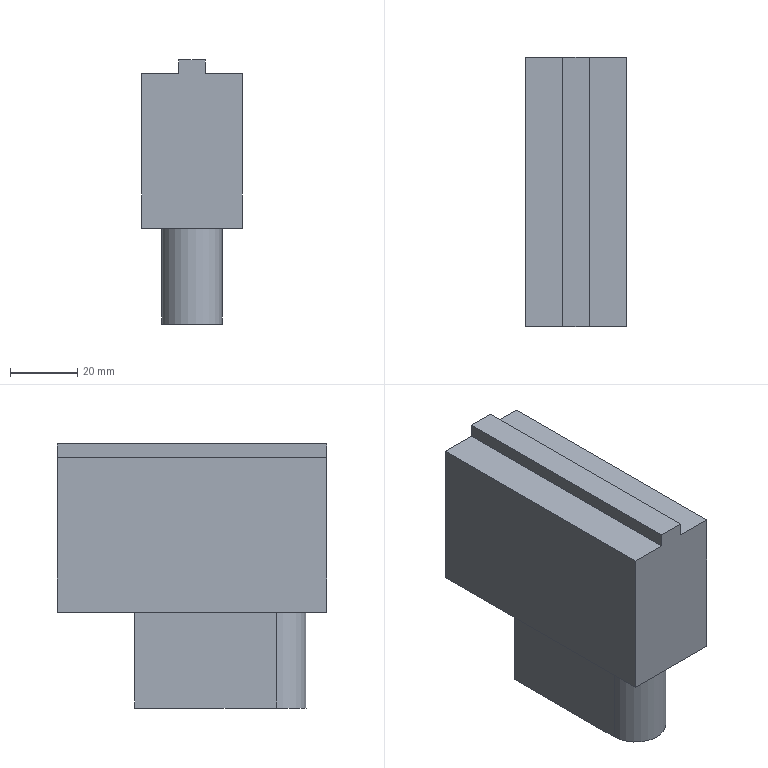Component | SolidWorks | 12AOuterSideWheel-EngravingAndMillingAxis-1_12AOuterSideWheelSeat-1 | 1 solid | 29 faces | box 30 x 80 x 78.5 mm | volume 131688 mm3 | plane 17 | cylinder 8 | cone 4 | commonest cylinder face diameters 8.5 x4 12.5 x3 18 x1 | material Cr12MoV
build123d program:
from build123d import *

# Parameters (mm, degrees)
SKETCH1_W              = 80
SKETCH1_H              = 46
BOSS_EXTRUDE1_DEPTH    = 30
SKETCH2_W              = 80
SKETCH2_H              = 8
BOSS_EXTRUDE2_DEPTH    = 4
BOSS_EXTRUDE3_DEPTH    = 28.5
M10_TAPPED_HOLE1_D     = 8.5
M10_TAPPED_HOLE1_DEPTH = 25
M10_TAPPED_HOLE1_TIP   = 2.554
CUT_EXTRUDE1_DEPTH     = 24


with BuildPart() as part:
    # Sketch1 → Boss-Extrude1 (new body)
    with BuildSketch(Plane.XY):
        with Locations((40, -23)):
            Rectangle(SKETCH1_W, SKETCH1_H)
    extrude(amount=BOSS_EXTRUDE1_DEPTH)

    # Sketch2 → Boss-Extrude2 (add)
    with BuildSketch(Plane(origin=(0, 0, 0), x_dir=(1, 0, 0), z_dir=(0, 1, 0))):
        with Locations((40, -15)):
            Rectangle(SKETCH2_W, SKETCH2_H)
    extrude(amount=BOSS_EXTRUDE2_DEPTH)

    # Sketch3 → Boss-Extrude3 (add)
    with BuildSketch(Plane.XZ.offset(46)):
        with BuildLine():
            Line((57, 24), (57, 6))
            Line((57, 6), (15, 6))
            ThreePointArc((15, 6), (6, 15), (15, 24))
            Line((15, 24), (57, 24))
        make_face()
    extrude(amount=BOSS_EXTRUDE3_DEPTH)

    # M10 Tapped Hole1
    with Locations(Plane(origin=(0, -74.5, 0), x_dir=(-1, 0, 0), z_dir=(0, -1, 0))):
        with Locations((-35, -15), (-15, -15)):
            Hole(M10_TAPPED_HOLE1_D / 2, depth=M10_TAPPED_HOLE1_DEPTH)
            with Locations((0, 0, -(M10_TAPPED_HOLE1_DEPTH + M10_TAPPED_HOLE1_TIP / 2))):  # 118° drill point
                Cone(0, M10_TAPPED_HOLE1_D / 2, M10_TAPPED_HOLE1_TIP, mode=Mode.SUBTRACT)

    # Sketch6 → Cut-Extrude1 (cut)
    with BuildSketch(Plane.XZ.offset(74.5)):
        with BuildLine():
            Line((57, 19.25), (53.083, 19.25))
            ThreePointArc((53.083, 19.25), (42.25, 15), (53.083, 10.75))
            Line((53.083, 10.75), (57, 10.75))
            Line((57, 10.75), (57, 19.25))
        make_face()
    extrude(amount=-CUT_EXTRUDE1_DEPTH, mode=Mode.SUBTRACT)


solid = part.part

# Placed as in the assembly
solid = solid.moved(Location((196.598, 111.538, 60.25), (90, 90, 0)))
STEP:
#1=COLOUR_RGB('',0.7922,0.8196,0.9333);
#2=FILL_AREA_STYLE_COLOUR('',#1);
#3=FILL_AREA_STYLE('',(#2));
#4=SURFACE_STYLE_FILL_AREA(#3);
#5=SURFACE_SIDE_STYLE('',(#4));
#6=SURFACE_STYLE_USAGE(.BOTH.,#5);
#7=PRESENTATION_STYLE_ASSIGNMENT((#6));
#8=CARTESIAN_POINT('',(8.577,6.301,0.3839));
#9=VERTEX_POINT('',#8);
#10=CARTESIAN_POINT('',(8.085,6.301,0.3839));
#11=VERTEX_POINT('',#10);
#12=CARTESIAN_POINT('',(8.331,6.301,0.3839));
#13=DIRECTION('',(0.,0.,-1.));
#14=DIRECTION('',(-1.,0.,0.));
#15=AXIS2_PLACEMENT_3D('',#12,#13,#14);
#16=CIRCLE('',#15,0.2461);
#17=EDGE_CURVE('',#9,#11,#16,.T.);
#18=ORIENTED_EDGE('',*,*,#17,.F.);
#19=CARTESIAN_POINT('',(8.577,6.301,-0.561));
#20=VERTEX_POINT('',#19);
#21=CARTESIAN_POINT('',(8.577,6.301,0.3839));
#22=DIRECTION('',(0.,0.,-1.));
#23=VECTOR('',#22,39.37);
#24=LINE('',#21,#23);
#25=EDGE_CURVE('',#9,#20,#24,.T.);
#26=ORIENTED_EDGE('',*,*,#25,.T.);
#27=CARTESIAN_POINT('',(8.085,6.301,-0.561));
#28=VERTEX_POINT('',#27);
#29=CARTESIAN_POINT('',(8.331,6.301,-0.561));
#30=DIRECTION('',(0.,0.,-1.));
#31=DIRECTION('',(-1.,0.,0.));
#32=AXIS2_PLACEMENT_3D('',#29,#30,#31);
#33=CIRCLE('',#32,0.2461);
#34=EDGE_CURVE('',#20,#28,#33,.T.);
#35=ORIENTED_EDGE('',*,*,#34,.T.);
#36=CARTESIAN_POINT('',(8.085,6.301,0.3839));
#37=DIRECTION('',(0.,0.,-1.));
#38=VECTOR('',#37,39.37);
#39=LINE('',#36,#38);
#40=EDGE_CURVE('',#11,#28,#39,.T.);
#41=ORIENTED_EDGE('',*,*,#40,.F.);
#42=EDGE_LOOP('',(#18,#26,#35,#41));
#43=FACE_OUTER_BOUND('',#42,.T.);
#44=CARTESIAN_POINT('',(8.331,6.301,0.3839));
#45=DIRECTION('',(0.,0.,-1.));
#46=DIRECTION('',(-1.,0.,0.));
#47=AXIS2_PLACEMENT_3D('',#44,#45,#46);
#48=CYLINDRICAL_SURFACE('',#47,0.2461);
#49=ADVANCED_FACE('',(#43),#48,.F.);
#50=CARTESIAN_POINT('',(8.163,6.481,0.3839));
#51=VERTEX_POINT('',#50);
#52=CARTESIAN_POINT('',(8.331,6.301,0.3839));
#53=DIRECTION('',(0.,0.,-1.));
#54=DIRECTION('',(-1.,0.,0.));
#55=AXIS2_PLACEMENT_3D('',#52,#53,#54);
#56=CIRCLE('',#55,0.2461);
#57=EDGE_CURVE('',#11,#51,#56,.T.);
#58=ORIENTED_EDGE('',*,*,#57,.F.);
#59=ORIENTED_EDGE('',*,*,#40,.T.);
#60=CARTESIAN_POINT('',(8.163,6.481,-0.561));
#61=VERTEX_POINT('',#60);
#62=CARTESIAN_POINT('',(8.331,6.301,-0.561));
#63=DIRECTION('',(0.,0.,-1.));
#64=DIRECTION('',(-1.,0.,0.));
#65=AXIS2_PLACEMENT_3D('',#62,#63,#64);
#66=CIRCLE('',#65,0.2461);
#67=EDGE_CURVE('',#28,#61,#66,.T.);
#68=ORIENTED_EDGE('',*,*,#67,.T.);
#69=CARTESIAN_POINT('',(8.163,6.481,0.3839));
#70=DIRECTION('',(0.,0.,-1.));
#71=VECTOR('',#70,39.37);
#72=LINE('',#69,#71);
#73=EDGE_CURVE('',#51,#61,#72,.T.);
#74=ORIENTED_EDGE('',*,*,#73,.F.);
#75=EDGE_LOOP('',(#58,#59,#68,#74));
#76=FACE_OUTER_BOUND('',#75,.T.);
#77=CARTESIAN_POINT('',(8.331,6.301,0.3839));
#78=DIRECTION('',(0.,0.,-1.));
#79=DIRECTION('',(-1.,0.,0.));
#80=AXIS2_PLACEMENT_3D('',#77,#78,#79);
#81=CYLINDRICAL_SURFACE('',#80,0.2461);
#82=ADVANCED_FACE('',(#76),#81,.F.);
#83=CARTESIAN_POINT('',(8.498,4.982,0.4232));
#84=VERTEX_POINT('',#83);
#85=CARTESIAN_POINT('',(8.163,4.982,0.4232));
#86=VERTEX_POINT('',#85);
#87=CARTESIAN_POINT('',(8.331,4.982,0.4232));
#88=DIRECTION('',(0.,0.,-1.));
#89=DIRECTION('',(-1.,0.,0.));
#90=AXIS2_PLACEMENT_3D('',#87,#88,#89);
#91=CIRCLE('',#90,0.1673);
#92=EDGE_CURVE('',#84,#86,#91,.T.);
#93=ORIENTED_EDGE('',*,*,#92,.F.);
#94=CARTESIAN_POINT('',(8.498,4.982,-0.561));
#95=VERTEX_POINT('',#94);
#96=CARTESIAN_POINT('',(8.498,4.982,-0.561));
#97=DIRECTION('',(0.,0.,-1.));
#98=VECTOR('',#97,39.37);
#99=LINE('',#96,#98);
#100=EDGE_CURVE('',#84,#95,#99,.T.);
#101=ORIENTED_EDGE('',*,*,#100,.T.);
#102=CARTESIAN_POINT('',(8.163,4.982,-0.561));
#103=VERTEX_POINT('',#102);
#104=CARTESIAN_POINT('',(8.331,4.982,-0.561));
#105=DIRECTION('',(0.,0.,-1.));
#106=DIRECTION('',(-1.,0.,0.));
#107=AXIS2_PLACEMENT_3D('',#104,#105,#106);
#108=CIRCLE('',#107,0.1673);
#109=EDGE_CURVE('',#95,#103,#108,.T.);
#110=ORIENTED_EDGE('',*,*,#109,.T.);
#111=CARTESIAN_POINT('',(8.163,4.982,-0.561));
#112=DIRECTION('',(0.,0.,-1.));
#113=VECTOR('',#112,39.37);
#114=LINE('',#111,#113);
#115=EDGE_CURVE('',#86,#103,#114,.T.);
#116=ORIENTED_EDGE('',*,*,#115,.F.);
#117=EDGE_LOOP('',(#93,#101,#110,#116));
#118=FACE_OUTER_BOUND('',#117,.T.);
#119=CARTESIAN_POINT('',(8.331,4.982,-0.561));
#120=DIRECTION('',(0.,0.,-1.));
#121=DIRECTION('',(-1.,0.,0.));
#122=AXIS2_PLACEMENT_3D('',#119,#120,#121);
#123=CYLINDRICAL_SURFACE('',#122,0.1673);
#124=ADVANCED_FACE('',(#118),#123,.F.);
#125=CARTESIAN_POINT('',(8.331,4.982,0.5238));
#126=VERTEX_POINT('',#125);
#127=CARTESIAN_POINT('',(8.163,4.982,0.4232));
#128=DIRECTION('',(-0.8572,0.,-0.515));
#129=VECTOR('',#128,39.37);
#130=LINE('',#127,#129);
#131=EDGE_CURVE('',#126,#86,#130,.T.);
#132=ORIENTED_EDGE('',*,*,#131,.F.);
#133=CARTESIAN_POINT('',(8.498,4.982,0.4232));
#134=DIRECTION('',(0.8572,0.,-0.515));
#135=VECTOR('',#134,39.37);
#136=LINE('',#133,#135);
#137=EDGE_CURVE('',#126,#84,#136,.T.);
#138=ORIENTED_EDGE('',*,*,#137,.T.);
#139=ORIENTED_EDGE('',*,*,#92,.T.);
#140=EDGE_LOOP('',(#132,#138,#139));
#141=FACE_OUTER_BOUND('',#140,.T.);
#142=CARTESIAN_POINT('',(8.331,4.982,0.4232));
#143=DIRECTION('',(0.,0.,-1.));
#144=DIRECTION('',(-1.,0.,0.));
#145=AXIS2_PLACEMENT_3D('',#142,#143,#144);
#146=CONICAL_SURFACE('',#145,0.1673,1.03);
#147=ADVANCED_FACE('',(#141),#146,.F.);
#148=CARTESIAN_POINT('',(8.498,5.769,0.4232));
#149=VERTEX_POINT('',#148);
#150=CARTESIAN_POINT('',(8.163,5.769,0.4232));
#151=VERTEX_POINT('',#150);
#152=CARTESIAN_POINT('',(8.331,5.769,0.4232));
#153=DIRECTION('',(0.,0.,-1.));
#154=DIRECTION('',(-1.,0.,0.));
#155=AXIS2_PLACEMENT_3D('',#152,#153,#154);
#156=CIRCLE('',#155,0.1673);
#157=EDGE_CURVE('',#149,#151,#156,.T.);
#158=ORIENTED_EDGE('',*,*,#157,.F.);
#159=CARTESIAN_POINT('',(8.498,5.769,-0.561));
#160=VERTEX_POINT('',#159);
#161=CARTESIAN_POINT('',(8.498,5.769,-0.561));
#162=DIRECTION('',(0.,0.,-1.));
#163=VECTOR('',#162,39.37);
#164=LINE('',#161,#163);
#165=EDGE_CURVE('',#149,#160,#164,.T.);
#166=ORIENTED_EDGE('',*,*,#165,.T.);
#167=CARTESIAN_POINT('',(8.163,5.769,-0.561));
#168=VERTEX_POINT('',#167);
#169=CARTESIAN_POINT('',(8.331,5.769,-0.561));
#170=DIRECTION('',(0.,0.,-1.));
#171=DIRECTION('',(-1.,0.,0.));
#172=AXIS2_PLACEMENT_3D('',#169,#170,#171);
#173=CIRCLE('',#172,0.1673);
#174=EDGE_CURVE('',#160,#168,#173,.T.);
#175=ORIENTED_EDGE('',*,*,#174,.T.);
#176=CARTESIAN_POINT('',(8.163,5.769,-0.561));
#177=DIRECTION('',(0.,0.,-1.));
#178=VECTOR('',#177,39.37);
#179=LINE('',#176,#178);
#180=EDGE_CURVE('',#151,#168,#179,.T.);
#181=ORIENTED_EDGE('',*,*,#180,.F.);
#182=EDGE_LOOP('',(#158,#166,#175,#181));
#183=FACE_OUTER_BOUND('',#182,.T.);
#184=CARTESIAN_POINT('',(8.331,5.769,-0.561));
#185=DIRECTION('',(0.,0.,-1.));
#186=DIRECTION('',(-1.,0.,0.));
#187=AXIS2_PLACEMENT_3D('',#184,#185,#186);
#188=CYLINDRICAL_SURFACE('',#187,0.1673);
#189=ADVANCED_FACE('',(#183),#188,.F.);
#190=CARTESIAN_POINT('',(8.331,5.769,0.5238));
#191=VERTEX_POINT('',#190);
#192=CARTESIAN_POINT('',(8.163,5.769,0.4232));
#193=DIRECTION('',(-0.8572,0.,-0.515));
#194=VECTOR('',#193,39.37);
#195=LINE('',#192,#194);
#196=EDGE_CURVE('',#191,#151,#195,.T.);
#197=ORIENTED_EDGE('',*,*,#196,.F.);
#198=CARTESIAN_POINT('',(8.498,5.769,0.4232));
#199=DIRECTION('',(0.8572,0.,-0.515));
#200=VECTOR('',#199,39.37);
#201=LINE('',#198,#200);
#202=EDGE_CURVE('',#191,#149,#201,.T.);
#203=ORIENTED_EDGE('',*,*,#202,.T.);
#204=ORIENTED_EDGE('',*,*,#157,.T.);
#205=EDGE_LOOP('',(#197,#203,#204));
#206=FACE_OUTER_BOUND('',#205,.T.);
#207=CARTESIAN_POINT('',(8.331,5.769,0.4232));
#208=DIRECTION('',(0.,0.,-1.));
#209=DIRECTION('',(-1.,0.,0.));
#210=AXIS2_PLACEMENT_3D('',#207,#208,#209);
#211=CONICAL_SURFACE('',#210,0.1673,1.03);
#212=ADVANCED_FACE('',(#206),#211,.F.);
#213=CARTESIAN_POINT('',(7.74,4.391,0.561));
#214=VERTEX_POINT('',#213);
#215=CARTESIAN_POINT('',(7.74,7.541,0.561));
#216=VERTEX_POINT('',#215);
#217=CARTESIAN_POINT('',(7.74,4.391,0.561));
#218=DIRECTION('',(0.,1.,0.));
#219=VECTOR('',#218,39.37);
#220=LINE('',#217,#219);
#221=EDGE_CURVE('',#214,#216,#220,.T.);
#222=ORIENTED_EDGE('',*,*,#221,.T.);
#223=CARTESIAN_POINT('',(8.921,7.541,0.561));
#224=VERTEX_POINT('',#223);
#225=CARTESIAN_POINT('',(8.921,7.541,0.561));
#226=DIRECTION('',(-1.,0.,0.));
#227=VECTOR('',#226,39.37);
#228=LINE('',#225,#227);
#229=EDGE_CURVE('',#224,#216,#228,.T.);
#230=ORIENTED_EDGE('',*,*,#229,.F.);
#231=CARTESIAN_POINT('',(8.921,4.391,0.561));
#232=VERTEX_POINT('',#231);
#233=CARTESIAN_POINT('',(8.921,4.391,0.561));
#234=DIRECTION('',(0.,1.,0.));
#235=VECTOR('',#234,39.37);
#236=LINE('',#233,#235);
#237=EDGE_CURVE('',#232,#224,#236,.T.);
#238=ORIENTED_EDGE('',*,*,#237,.F.);
#239=CARTESIAN_POINT('',(8.921,4.391,0.561));
#240=DIRECTION('',(-1.,0.,0.));
#241=VECTOR('',#240,39.37);
#242=LINE('',#239,#241);
#243=EDGE_CURVE('',#232,#214,#242,.T.);
#244=ORIENTED_EDGE('',*,*,#243,.T.);
#245=EDGE_LOOP('',(#222,#230,#238,#244));
#246=FACE_OUTER_BOUND('',#245,.T.);
#247=CARTESIAN_POINT('',(8.685,4.982,0.561));
#248=VERTEX_POINT('',#247);
#249=CARTESIAN_POINT('',(7.976,4.982,0.561));
#250=VERTEX_POINT('',#249);
#251=CARTESIAN_POINT('',(8.331,4.982,0.561));
#252=DIRECTION('',(0.,0.,-1.));
#253=DIRECTION('',(-1.,0.,0.));
#254=AXIS2_PLACEMENT_3D('',#251,#252,#253);
#255=CIRCLE('',#254,0.3543);
#256=EDGE_CURVE('',#248,#250,#255,.T.);
#257=ORIENTED_EDGE('',*,*,#256,.F.);
#258=CARTESIAN_POINT('',(8.685,6.635,0.561));
#259=VERTEX_POINT('',#258);
#260=CARTESIAN_POINT('',(8.685,4.982,0.561));
#261=DIRECTION('',(0.,-1.,0.));
#262=VECTOR('',#261,39.37);
#263=LINE('',#260,#262);
#264=EDGE_CURVE('',#259,#248,#263,.T.);
#265=ORIENTED_EDGE('',*,*,#264,.F.);
#266=CARTESIAN_POINT('',(7.976,6.635,0.561));
#267=VERTEX_POINT('',#266);
#268=CARTESIAN_POINT('',(8.685,6.635,0.561));
#269=DIRECTION('',(1.,0.,0.));
#270=VECTOR('',#269,39.37);
#271=LINE('',#268,#270);
#272=EDGE_CURVE('',#267,#259,#271,.T.);
#273=ORIENTED_EDGE('',*,*,#272,.F.);
#274=CARTESIAN_POINT('',(7.976,4.982,0.561));
#275=DIRECTION('',(0.,1.,0.));
#276=VECTOR('',#275,39.37);
#277=LINE('',#274,#276);
#278=EDGE_CURVE('',#250,#267,#277,.T.);
#279=ORIENTED_EDGE('',*,*,#278,.F.);
#280=EDGE_LOOP('',(#257,#265,#273,#279));
#281=FACE_BOUND('',#280,.T.);
#282=CARTESIAN_POINT('',(8.921,4.391,0.561));
#283=DIRECTION('',(0.,0.,1.));
#284=DIRECTION('',(1.,0.,0.));
#285=AXIS2_PLACEMENT_3D('',#282,#283,#284);
#286=PLANE('',#285);
#287=ADVANCED_FACE('',(#246,#281),#286,.F.);
#288=CARTESIAN_POINT('',(8.173,7.541,2.372));
#289=VERTEX_POINT('',#288);
#290=CARTESIAN_POINT('',(8.173,4.391,2.372));
#291=VERTEX_POINT('',#290);
#292=CARTESIAN_POINT('',(8.173,4.391,2.372));
#293=DIRECTION('',(0.,-1.,0.));
#294=VECTOR('',#293,39.37);
#295=LINE('',#292,#294);
#296=EDGE_CURVE('',#289,#291,#295,.T.);
#297=ORIENTED_EDGE('',*,*,#296,.F.);
#298=CARTESIAN_POINT('',(7.74,7.541,2.372));
#299=VERTEX_POINT('',#298);
#300=CARTESIAN_POINT('',(8.921,7.541,2.372));
#301=DIRECTION('',(-1.,0.,0.));
#302=VECTOR('',#301,39.37);
#303=LINE('',#300,#302);
#304=EDGE_CURVE('',#289,#299,#303,.T.);
#305=ORIENTED_EDGE('',*,*,#304,.T.);
#306=CARTESIAN_POINT('',(7.74,4.391,2.372));
#307=VERTEX_POINT('',#306);
#308=CARTESIAN_POINT('',(7.74,4.391,2.372));
#309=DIRECTION('',(0.,-1.,0.));
#310=VECTOR('',#309,39.37);
#311=LINE('',#308,#310);
#312=EDGE_CURVE('',#299,#307,#311,.T.);
#313=ORIENTED_EDGE('',*,*,#312,.T.);
#314=CARTESIAN_POINT('',(8.921,4.391,2.372));
#315=DIRECTION('',(-1.,0.,0.));
#316=VECTOR('',#315,39.37);
#317=LINE('',#314,#316);
#318=EDGE_CURVE('',#291,#307,#317,.T.);
#319=ORIENTED_EDGE('',*,*,#318,.F.);
#320=EDGE_LOOP('',(#297,#305,#313,#319));
#321=FACE_OUTER_BOUND('',#320,.T.);
#322=CARTESIAN_POINT('',(8.921,4.391,2.372));
#323=DIRECTION('',(0.,0.,-1.));
#324=DIRECTION('',(-1.,0.,0.));
#325=AXIS2_PLACEMENT_3D('',#322,#323,#324);
#326=PLANE('',#325);
#327=ADVANCED_FACE('',(#321),#326,.F.);
#328=CARTESIAN_POINT('',(8.488,4.391,2.372));
#329=VERTEX_POINT('',#328);
#330=CARTESIAN_POINT('',(8.488,7.541,2.372));
#331=VERTEX_POINT('',#330);
#332=CARTESIAN_POINT('',(8.488,4.391,2.372));
#333=DIRECTION('',(-0.,1.,0.));
#334=VECTOR('',#333,39.37);
#335=LINE('',#332,#334);
#336=EDGE_CURVE('',#329,#331,#335,.T.);
#337=ORIENTED_EDGE('',*,*,#336,.F.);
#338=CARTESIAN_POINT('',(8.921,4.391,2.372));
#339=VERTEX_POINT('',#338);
#340=CARTESIAN_POINT('',(8.921,4.391,2.372));
#341=DIRECTION('',(-1.,0.,0.));
#342=VECTOR('',#341,39.37);
#343=LINE('',#340,#342);
#344=EDGE_CURVE('',#339,#329,#343,.T.);
#345=ORIENTED_EDGE('',*,*,#344,.F.);
#346=CARTESIAN_POINT('',(8.921,7.541,2.372));
#347=VERTEX_POINT('',#346);
#348=CARTESIAN_POINT('',(8.921,4.391,2.372));
#349=DIRECTION('',(0.,-1.,0.));
#350=VECTOR('',#349,39.37);
#351=LINE('',#348,#350);
#352=EDGE_CURVE('',#347,#339,#351,.T.);
#353=ORIENTED_EDGE('',*,*,#352,.F.);
#354=CARTESIAN_POINT('',(8.921,7.541,2.372));
#355=DIRECTION('',(-1.,0.,0.));
#356=VECTOR('',#355,39.37);
#357=LINE('',#354,#356);
#358=EDGE_CURVE('',#347,#331,#357,.T.);
#359=ORIENTED_EDGE('',*,*,#358,.T.);
#360=EDGE_LOOP('',(#337,#345,#353,#359));
#361=FACE_OUTER_BOUND('',#360,.T.);
#362=CARTESIAN_POINT('',(8.921,4.391,2.372));
#363=DIRECTION('',(0.,0.,-1.));
#364=DIRECTION('',(-1.,0.,0.));
#365=AXIS2_PLACEMENT_3D('',#362,#363,#364);
#366=PLANE('',#365);
#367=ADVANCED_FACE('',(#361),#366,.F.);
#368=CARTESIAN_POINT('',(7.74,4.391,2.372));
#369=DIRECTION('',(0.,0.,-1.));
#370=VECTOR('',#369,39.37);
#371=LINE('',#368,#370);
#372=EDGE_CURVE('',#307,#214,#371,.T.);
#373=ORIENTED_EDGE('',*,*,#372,.T.);
#374=ORIENTED_EDGE('',*,*,#243,.F.);
#375=CARTESIAN_POINT('',(8.921,4.391,2.372));
#376=DIRECTION('',(0.,0.,-1.));
#377=VECTOR('',#376,39.37);
#378=LINE('',#375,#377);
#379=EDGE_CURVE('',#339,#232,#378,.T.);
#380=ORIENTED_EDGE('',*,*,#379,.F.);
#381=ORIENTED_EDGE('',*,*,#344,.T.);
#382=CARTESIAN_POINT('',(8.488,4.391,2.53));
#383=VERTEX_POINT('',#382);
#384=CARTESIAN_POINT('',(8.488,4.391,2.53));
#385=DIRECTION('',(0.,0.,-1.));
#386=VECTOR('',#385,39.37);
#387=LINE('',#384,#386);
#388=EDGE_CURVE('',#383,#329,#387,.T.);
#389=ORIENTED_EDGE('',*,*,#388,.F.);
#390=CARTESIAN_POINT('',(8.173,4.391,2.53));
#391=VERTEX_POINT('',#390);
#392=CARTESIAN_POINT('',(8.173,4.391,2.53));
#393=DIRECTION('',(1.,0.,0.));
#394=VECTOR('',#393,39.37);
#395=LINE('',#392,#394);
#396=EDGE_CURVE('',#391,#383,#395,.T.);
#397=ORIENTED_EDGE('',*,*,#396,.F.);
#398=CARTESIAN_POINT('',(8.173,4.391,2.53));
#399=DIRECTION('',(0.,0.,-1.));
#400=VECTOR('',#399,39.37);
#401=LINE('',#398,#400);
#402=EDGE_CURVE('',#391,#291,#401,.T.);
#403=ORIENTED_EDGE('',*,*,#402,.T.);
#404=ORIENTED_EDGE('',*,*,#318,.T.);
#405=EDGE_LOOP('',(#373,#374,#380,#381,#389,#397,#403,#404));
#406=FACE_OUTER_BOUND('',#405,.T.);
#407=CARTESIAN_POINT('',(8.921,4.391,2.372));
#408=DIRECTION('',(0.,1.,0.));
#409=DIRECTION('',(0.,-0.,1.));
#410=AXIS2_PLACEMENT_3D('',#407,#408,#409);
#411=PLANE('',#410);
#412=ADVANCED_FACE('',(#406),#411,.F.);
#413=CARTESIAN_POINT('',(7.74,7.541,2.372));
#414=DIRECTION('',(0.,-0.,1.));
#415=VECTOR('',#414,39.37);
#416=LINE('',#413,#415);
#417=EDGE_CURVE('',#216,#299,#416,.T.);
#418=ORIENTED_EDGE('',*,*,#417,.T.);
#419=ORIENTED_EDGE('',*,*,#304,.F.);
#420=CARTESIAN_POINT('',(8.173,7.541,2.53));
#421=VERTEX_POINT('',#420);
#422=CARTESIAN_POINT('',(8.173,7.541,2.53));
#423=DIRECTION('',(0.,0.,-1.));
#424=VECTOR('',#423,39.37);
#425=LINE('',#422,#424);
#426=EDGE_CURVE('',#421,#289,#425,.T.);
#427=ORIENTED_EDGE('',*,*,#426,.F.);
#428=CARTESIAN_POINT('',(8.488,7.541,2.53));
#429=VERTEX_POINT('',#428);
#430=CARTESIAN_POINT('',(8.173,7.541,2.53));
#431=DIRECTION('',(-1.,0.,0.));
#432=VECTOR('',#431,39.37);
#433=LINE('',#430,#432);
#434=EDGE_CURVE('',#429,#421,#433,.T.);
#435=ORIENTED_EDGE('',*,*,#434,.F.);
#436=CARTESIAN_POINT('',(8.488,7.541,2.53));
#437=DIRECTION('',(0.,0.,-1.));
#438=VECTOR('',#437,39.37);
#439=LINE('',#436,#438);
#440=EDGE_CURVE('',#429,#331,#439,.T.);
#441=ORIENTED_EDGE('',*,*,#440,.T.);
#442=ORIENTED_EDGE('',*,*,#358,.F.);
#443=CARTESIAN_POINT('',(8.921,7.541,2.372));
#444=DIRECTION('',(0.,-0.,1.));
#445=VECTOR('',#444,39.37);
#446=LINE('',#443,#445);
#447=EDGE_CURVE('',#224,#347,#446,.T.);
#448=ORIENTED_EDGE('',*,*,#447,.F.);
#449=ORIENTED_EDGE('',*,*,#229,.T.);
#450=EDGE_LOOP('',(#418,#419,#427,#435,#441,#442,#448,#449));
#451=FACE_OUTER_BOUND('',#450,.T.);
#452=CARTESIAN_POINT('',(8.921,7.541,2.372));
#453=DIRECTION('',(0.,-1.,-0.));
#454=DIRECTION('',(0.,0.,-1.));
#455=AXIS2_PLACEMENT_3D('',#452,#453,#454);
#456=PLANE('',#455);
#457=ADVANCED_FACE('',(#451),#456,.F.);
#458=ORIENTED_EDGE('',*,*,#379,.T.);
#459=ORIENTED_EDGE('',*,*,#237,.T.);
#460=ORIENTED_EDGE('',*,*,#447,.T.);
#461=ORIENTED_EDGE('',*,*,#352,.T.);
#462=EDGE_LOOP('',(#458,#459,#460,#461));
#463=FACE_OUTER_BOUND('',#462,.T.);
#464=CARTESIAN_POINT('',(8.921,4.391,2.372));
#465=DIRECTION('',(1.,0.,0.));
#466=DIRECTION('',(0.,1.,0.));
#467=AXIS2_PLACEMENT_3D('',#464,#465,#466);
#468=PLANE('',#467);
#469=ADVANCED_FACE('',(#463),#468,.T.);
#470=ORIENTED_EDGE('',*,*,#372,.F.);
#471=ORIENTED_EDGE('',*,*,#312,.F.);
#472=ORIENTED_EDGE('',*,*,#417,.F.);
#473=ORIENTED_EDGE('',*,*,#221,.F.);
#474=EDGE_LOOP('',(#470,#471,#472,#473));
#475=FACE_OUTER_BOUND('',#474,.T.);
#476=CARTESIAN_POINT('',(7.74,4.391,2.372));
#477=DIRECTION('',(1.,0.,0.));
#478=DIRECTION('',(0.,1.,0.));
#479=AXIS2_PLACEMENT_3D('',#476,#477,#478);
#480=PLANE('',#479);
#481=ADVANCED_FACE('',(#475),#480,.F.);
#482=ORIENTED_EDGE('',*,*,#336,.T.);
#483=ORIENTED_EDGE('',*,*,#440,.F.);
#484=CARTESIAN_POINT('',(8.488,4.391,2.53));
#485=DIRECTION('',(-0.,1.,0.));
#486=VECTOR('',#485,39.37);
#487=LINE('',#484,#486);
#488=EDGE_CURVE('',#383,#429,#487,.T.);
#489=ORIENTED_EDGE('',*,*,#488,.F.);
#490=ORIENTED_EDGE('',*,*,#388,.T.);
#491=EDGE_LOOP('',(#482,#483,#489,#490));
#492=FACE_OUTER_BOUND('',#491,.T.);
#493=CARTESIAN_POINT('',(8.488,4.391,2.53));
#494=DIRECTION('',(-1.,-0.,0.));
#495=DIRECTION('',(0.,-1.,0.));
#496=AXIS2_PLACEMENT_3D('',#493,#494,#495);
#497=PLANE('',#496);
#498=ADVANCED_FACE('',(#492),#497,.F.);
#499=ORIENTED_EDGE('',*,*,#296,.T.);
#500=ORIENTED_EDGE('',*,*,#402,.F.);
#501=CARTESIAN_POINT('',(8.173,4.391,2.53));
#502=DIRECTION('',(0.,-1.,0.));
#503=VECTOR('',#502,39.37);
#504=LINE('',#501,#503);
#505=EDGE_CURVE('',#421,#391,#504,.T.);
#506=ORIENTED_EDGE('',*,*,#505,.F.);
#507=ORIENTED_EDGE('',*,*,#426,.T.);
#508=EDGE_LOOP('',(#499,#500,#506,#507));
#509=FACE_OUTER_BOUND('',#508,.T.);
#510=CARTESIAN_POINT('',(8.173,4.391,2.53));
#511=DIRECTION('',(1.,0.,0.));
#512=DIRECTION('',(0.,1.,0.));
#513=AXIS2_PLACEMENT_3D('',#510,#511,#512);
#514=PLANE('',#513);
#515=ADVANCED_FACE('',(#509),#514,.F.);
#516=ORIENTED_EDGE('',*,*,#396,.T.);
#517=ORIENTED_EDGE('',*,*,#488,.T.);
#518=ORIENTED_EDGE('',*,*,#434,.T.);
#519=ORIENTED_EDGE('',*,*,#505,.T.);
#520=EDGE_LOOP('',(#516,#517,#518,#519));
#521=FACE_OUTER_BOUND('',#520,.T.);
#522=CARTESIAN_POINT('',(7.74,4.391,2.53));
#523=DIRECTION('',(0.,0.,1.));
#524=DIRECTION('',(1.,0.,0.));
#525=AXIS2_PLACEMENT_3D('',#522,#523,#524);
#526=PLANE('',#525);
#527=ADVANCED_FACE('',(#521),#526,.T.);
#528=ORIENTED_EDGE('',*,*,#256,.T.);
#529=CARTESIAN_POINT('',(7.976,4.982,-0.561));
#530=VERTEX_POINT('',#529);
#531=CARTESIAN_POINT('',(7.976,4.982,-0.561));
#532=DIRECTION('',(0.,0.,1.));
#533=VECTOR('',#532,39.37);
#534=LINE('',#531,#533);
#535=EDGE_CURVE('',#530,#250,#534,.T.);
#536=ORIENTED_EDGE('',*,*,#535,.F.);
#537=CARTESIAN_POINT('',(8.685,4.982,-0.561));
#538=VERTEX_POINT('',#537);
#539=CARTESIAN_POINT('',(8.331,4.982,-0.561));
#540=DIRECTION('',(0.,0.,-1.));
#541=DIRECTION('',(-1.,0.,0.));
#542=AXIS2_PLACEMENT_3D('',#539,#540,#541);
#543=CIRCLE('',#542,0.3543);
#544=EDGE_CURVE('',#538,#530,#543,.T.);
#545=ORIENTED_EDGE('',*,*,#544,.F.);
#546=CARTESIAN_POINT('',(8.685,4.982,-0.561));
#547=DIRECTION('',(0.,0.,1.));
#548=VECTOR('',#547,39.37);
#549=LINE('',#546,#548);
#550=EDGE_CURVE('',#538,#248,#549,.T.);
#551=ORIENTED_EDGE('',*,*,#550,.T.);
#552=EDGE_LOOP('',(#528,#536,#545,#551));
#553=FACE_OUTER_BOUND('',#552,.T.);
#554=CARTESIAN_POINT('',(8.331,4.982,-0.561));
#555=DIRECTION('',(0.,0.,1.));
#556=DIRECTION('',(1.,0.,0.));
#557=AXIS2_PLACEMENT_3D('',#554,#555,#556);
#558=CYLINDRICAL_SURFACE('',#557,0.3543);
#559=ADVANCED_FACE('',(#553),#558,.T.);
#560=ORIENTED_EDGE('',*,*,#278,.T.);
#561=CARTESIAN_POINT('',(7.976,6.635,-0.561));
#562=VERTEX_POINT('',#561);
#563=CARTESIAN_POINT('',(7.976,6.635,-0.561));
#564=DIRECTION('',(0.,0.,1.));
#565=VECTOR('',#564,39.37);
#566=LINE('',#563,#565);
#567=EDGE_CURVE('',#562,#267,#566,.T.);
#568=ORIENTED_EDGE('',*,*,#567,.F.);
#569=CARTESIAN_POINT('',(7.976,4.982,-0.561));
#570=DIRECTION('',(0.,1.,0.));
#571=VECTOR('',#570,39.37);
#572=LINE('',#569,#571);
#573=EDGE_CURVE('',#530,#562,#572,.T.);
#574=ORIENTED_EDGE('',*,*,#573,.F.);
#575=ORIENTED_EDGE('',*,*,#535,.T.);
#576=EDGE_LOOP('',(#560,#568,#574,#575));
#577=FACE_OUTER_BOUND('',#576,.T.);
#578=CARTESIAN_POINT('',(7.976,4.982,-0.561));
#579=DIRECTION('',(1.,0.,0.));
#580=DIRECTION('',(0.,1.,0.));
#581=AXIS2_PLACEMENT_3D('',#578,#579,#580);
#582=PLANE('',#581);
#583=ADVANCED_FACE('',(#577),#582,.F.);
#584=CARTESIAN_POINT('',(8.163,6.635,0.3839));
#585=VERTEX_POINT('',#584);
#586=CARTESIAN_POINT('',(8.498,6.635,0.3839));
#587=VERTEX_POINT('',#586);
#588=CARTESIAN_POINT('',(8.498,6.635,0.3839));
#589=DIRECTION('',(1.,0.,0.));
#590=VECTOR('',#589,39.37);
#591=LINE('',#588,#590);
#592=EDGE_CURVE('',#585,#587,#591,.T.);
#593=ORIENTED_EDGE('',*,*,#592,.F.);
#594=CARTESIAN_POINT('',(8.163,6.635,-0.561));
#595=VERTEX_POINT('',#594);
#596=CARTESIAN_POINT('',(8.163,6.635,0.3839));
#597=DIRECTION('',(0.,0.,-1.));
#598=VECTOR('',#597,39.37);
#599=LINE('',#596,#598);
#600=EDGE_CURVE('',#585,#595,#599,.T.);
#601=ORIENTED_EDGE('',*,*,#600,.T.);
#602=CARTESIAN_POINT('',(8.685,6.635,-0.561));
#603=DIRECTION('',(1.,0.,0.));
#604=VECTOR('',#603,39.37);
#605=LINE('',#602,#604);
#606=EDGE_CURVE('',#562,#595,#605,.T.);
#607=ORIENTED_EDGE('',*,*,#606,.F.);
#608=ORIENTED_EDGE('',*,*,#567,.T.);
#609=ORIENTED_EDGE('',*,*,#272,.T.);
#610=CARTESIAN_POINT('',(8.685,6.635,-0.561));
#611=VERTEX_POINT('',#610);
#612=CARTESIAN_POINT('',(8.685,6.635,-0.561));
#613=DIRECTION('',(0.,0.,1.));
#614=VECTOR('',#613,39.37);
#615=LINE('',#612,#614);
#616=EDGE_CURVE('',#611,#259,#615,.T.);
#617=ORIENTED_EDGE('',*,*,#616,.F.);
#618=CARTESIAN_POINT('',(8.498,6.635,-0.561));
#619=VERTEX_POINT('',#618);
#620=CARTESIAN_POINT('',(8.685,6.635,-0.561));
#621=DIRECTION('',(1.,0.,0.));
#622=VECTOR('',#621,39.37);
#623=LINE('',#620,#622);
#624=EDGE_CURVE('',#619,#611,#623,.T.);
#625=ORIENTED_EDGE('',*,*,#624,.F.);
#626=CARTESIAN_POINT('',(8.498,6.635,0.3839));
#627=DIRECTION('',(0.,0.,-1.));
#628=VECTOR('',#627,39.37);
#629=LINE('',#626,#628);
#630=EDGE_CURVE('',#587,#619,#629,.T.);
#631=ORIENTED_EDGE('',*,*,#630,.F.);
#632=EDGE_LOOP('',(#593,#601,#607,#608,#609,#617,#625,#631));
#633=FACE_OUTER_BOUND('',#632,.T.);
#634=CARTESIAN_POINT('',(8.685,6.635,-0.561));
#635=DIRECTION('',(0.,-1.,0.));
#636=DIRECTION('',(1.,0.,0.));
#637=AXIS2_PLACEMENT_3D('',#634,#635,#636);
#638=PLANE('',#637);
#639=ADVANCED_FACE('',(#633),#638,.F.);
#640=ORIENTED_EDGE('',*,*,#264,.T.);
#641=ORIENTED_EDGE('',*,*,#550,.F.);
#642=CARTESIAN_POINT('',(8.685,4.982,-0.561));
#643=DIRECTION('',(0.,-1.,0.));
#644=VECTOR('',#643,39.37);
#645=LINE('',#642,#644);
#646=EDGE_CURVE('',#611,#538,#645,.T.);
#647=ORIENTED_EDGE('',*,*,#646,.F.);
#648=ORIENTED_EDGE('',*,*,#616,.T.);
#649=EDGE_LOOP('',(#640,#641,#647,#648));
#650=FACE_OUTER_BOUND('',#649,.T.);
#651=CARTESIAN_POINT('',(8.685,4.982,-0.561));
#652=DIRECTION('',(-1.,0.,0.));
#653=DIRECTION('',(0.,-1.,0.));
#654=AXIS2_PLACEMENT_3D('',#651,#652,#653);
#655=PLANE('',#654);
#656=ADVANCED_FACE('',(#650),#655,.F.);
#657=CARTESIAN_POINT('',(8.163,6.635,-0.561));
#658=DIRECTION('',(0.,1.,0.));
#659=VECTOR('',#658,39.37);
#660=LINE('',#657,#659);
#661=EDGE_CURVE('',#61,#595,#660,.T.);
#662=ORIENTED_EDGE('',*,*,#661,.F.);
#663=ORIENTED_EDGE('',*,*,#67,.F.);
#664=ORIENTED_EDGE('',*,*,#34,.F.);
#665=CARTESIAN_POINT('',(8.498,6.481,-0.561));
#666=VERTEX_POINT('',#665);
#667=CARTESIAN_POINT('',(8.331,6.301,-0.561));
#668=DIRECTION('',(0.,0.,-1.));
#669=DIRECTION('',(-1.,0.,0.));
#670=AXIS2_PLACEMENT_3D('',#667,#668,#669);
#671=CIRCLE('',#670,0.2461);
#672=EDGE_CURVE('',#666,#20,#671,.T.);
#673=ORIENTED_EDGE('',*,*,#672,.F.);
#674=CARTESIAN_POINT('',(8.498,6.635,-0.561));
#675=DIRECTION('',(0.,-1.,0.));
#676=VECTOR('',#675,39.37);
#677=LINE('',#674,#676);
#678=EDGE_CURVE('',#619,#666,#677,.T.);
#679=ORIENTED_EDGE('',*,*,#678,.F.);
#680=ORIENTED_EDGE('',*,*,#624,.T.);
#681=ORIENTED_EDGE('',*,*,#646,.T.);
#682=ORIENTED_EDGE('',*,*,#544,.T.);
#683=ORIENTED_EDGE('',*,*,#573,.T.);
#684=ORIENTED_EDGE('',*,*,#606,.T.);
#685=EDGE_LOOP('',(#662,#663,#664,#673,#679,#680,#681,#682,#683,#684));
#686=FACE_OUTER_BOUND('',#685,.T.);
#687=CARTESIAN_POINT('',(8.331,4.982,-0.561));
#688=DIRECTION('',(0.,0.,-1.));
#689=DIRECTION('',(-1.,0.,0.));
#690=AXIS2_PLACEMENT_3D('',#687,#688,#689);
#691=CIRCLE('',#690,0.1673);
#692=EDGE_CURVE('',#103,#95,#691,.T.);
#693=ORIENTED_EDGE('',*,*,#692,.F.);
#694=ORIENTED_EDGE('',*,*,#109,.F.);
#695=EDGE_LOOP('',(#693,#694));
#696=FACE_BOUND('',#695,.T.);
#697=CARTESIAN_POINT('',(8.331,5.769,-0.561));
#698=DIRECTION('',(0.,0.,-1.));
#699=DIRECTION('',(-1.,0.,0.));
#700=AXIS2_PLACEMENT_3D('',#697,#698,#699);
#701=CIRCLE('',#700,0.1673);
#702=EDGE_CURVE('',#168,#160,#701,.T.);
#703=ORIENTED_EDGE('',*,*,#702,.F.);
#704=ORIENTED_EDGE('',*,*,#174,.F.);
#705=EDGE_LOOP('',(#703,#704));
#706=FACE_BOUND('',#705,.T.);
#707=CARTESIAN_POINT('',(8.331,4.982,-0.561));
#708=DIRECTION('',(0.,0.,-1.));
#709=DIRECTION('',(-1.,0.,0.));
#710=AXIS2_PLACEMENT_3D('',#707,#708,#709);
#711=PLANE('',#710);
#712=ADVANCED_FACE('',(#686,#696,#706),#711,.T.);
#713=ORIENTED_EDGE('',*,*,#202,.F.);
#714=ORIENTED_EDGE('',*,*,#196,.T.);
#715=CARTESIAN_POINT('',(8.331,5.769,0.4232));
#716=DIRECTION('',(0.,0.,-1.));
#717=DIRECTION('',(-1.,0.,0.));
#718=AXIS2_PLACEMENT_3D('',#715,#716,#717);
#719=CIRCLE('',#718,0.1673);
#720=EDGE_CURVE('',#151,#149,#719,.T.);
#721=ORIENTED_EDGE('',*,*,#720,.T.);
#722=EDGE_LOOP('',(#713,#714,#721));
#723=FACE_OUTER_BOUND('',#722,.T.);
#724=CARTESIAN_POINT('',(8.331,5.769,0.4232));
#725=DIRECTION('',(0.,0.,-1.));
#726=DIRECTION('',(-1.,0.,0.));
#727=AXIS2_PLACEMENT_3D('',#724,#725,#726);
#728=CONICAL_SURFACE('',#727,0.1673,1.03);
#729=ADVANCED_FACE('',(#723),#728,.F.);
#730=ORIENTED_EDGE('',*,*,#165,.F.);
#731=ORIENTED_EDGE('',*,*,#720,.F.);
#732=ORIENTED_EDGE('',*,*,#180,.T.);
#733=ORIENTED_EDGE('',*,*,#702,.T.);
#734=EDGE_LOOP('',(#730,#731,#732,#733));
#735=FACE_OUTER_BOUND('',#734,.T.);
#736=CARTESIAN_POINT('',(8.331,5.769,-0.561));
#737=DIRECTION('',(0.,0.,-1.));
#738=DIRECTION('',(-1.,0.,0.));
#739=AXIS2_PLACEMENT_3D('',#736,#737,#738);
#740=CYLINDRICAL_SURFACE('',#739,0.1673);
#741=ADVANCED_FACE('',(#735),#740,.F.);
#742=ORIENTED_EDGE('',*,*,#137,.F.);
#743=ORIENTED_EDGE('',*,*,#131,.T.);
#744=CARTESIAN_POINT('',(8.331,4.982,0.4232));
#745=DIRECTION('',(0.,0.,-1.));
#746=DIRECTION('',(-1.,0.,0.));
#747=AXIS2_PLACEMENT_3D('',#744,#745,#746);
#748=CIRCLE('',#747,0.1673);
#749=EDGE_CURVE('',#86,#84,#748,.T.);
#750=ORIENTED_EDGE('',*,*,#749,.T.);
#751=EDGE_LOOP('',(#742,#743,#750));
#752=FACE_OUTER_BOUND('',#751,.T.);
#753=CARTESIAN_POINT('',(8.331,4.982,0.4232));
#754=DIRECTION('',(0.,0.,-1.));
#755=DIRECTION('',(-1.,0.,0.));
#756=AXIS2_PLACEMENT_3D('',#753,#754,#755);
#757=CONICAL_SURFACE('',#756,0.1673,1.03);
#758=ADVANCED_FACE('',(#752),#757,.F.);
#759=ORIENTED_EDGE('',*,*,#100,.F.);
#760=ORIENTED_EDGE('',*,*,#749,.F.);
#761=ORIENTED_EDGE('',*,*,#115,.T.);
#762=ORIENTED_EDGE('',*,*,#692,.T.);
#763=EDGE_LOOP('',(#759,#760,#761,#762));
#764=FACE_OUTER_BOUND('',#763,.T.);
#765=CARTESIAN_POINT('',(8.331,4.982,-0.561));
#766=DIRECTION('',(0.,0.,-1.));
#767=DIRECTION('',(-1.,0.,0.));
#768=AXIS2_PLACEMENT_3D('',#765,#766,#767);
#769=CYLINDRICAL_SURFACE('',#768,0.1673);
#770=ADVANCED_FACE('',(#764),#769,.F.);
#771=ORIENTED_EDGE('',*,*,#661,.T.);
#772=ORIENTED_EDGE('',*,*,#600,.F.);
#773=CARTESIAN_POINT('',(8.163,6.635,0.3839));
#774=DIRECTION('',(0.,1.,0.));
#775=VECTOR('',#774,39.37);
#776=LINE('',#773,#775);
#777=EDGE_CURVE('',#51,#585,#776,.T.);
#778=ORIENTED_EDGE('',*,*,#777,.F.);
#779=ORIENTED_EDGE('',*,*,#73,.T.);
#780=EDGE_LOOP('',(#771,#772,#778,#779));
#781=FACE_OUTER_BOUND('',#780,.T.);
#782=CARTESIAN_POINT('',(8.163,6.635,0.3839));
#783=DIRECTION('',(-1.,0.,0.));
#784=DIRECTION('',(0.,-1.,0.));
#785=AXIS2_PLACEMENT_3D('',#782,#783,#784);
#786=PLANE('',#785);
#787=ADVANCED_FACE('',(#781),#786,.F.);
#788=ORIENTED_EDGE('',*,*,#25,.F.);
#789=CARTESIAN_POINT('',(8.498,6.481,0.3839));
#790=VERTEX_POINT('',#789);
#791=CARTESIAN_POINT('',(8.331,6.301,0.3839));
#792=DIRECTION('',(0.,0.,-1.));
#793=DIRECTION('',(-1.,0.,0.));
#794=AXIS2_PLACEMENT_3D('',#791,#792,#793);
#795=CIRCLE('',#794,0.2461);
#796=EDGE_CURVE('',#790,#9,#795,.T.);
#797=ORIENTED_EDGE('',*,*,#796,.F.);
#798=CARTESIAN_POINT('',(8.498,6.481,0.3839));
#799=DIRECTION('',(0.,0.,-1.));
#800=VECTOR('',#799,39.37);
#801=LINE('',#798,#800);
#802=EDGE_CURVE('',#790,#666,#801,.T.);
#803=ORIENTED_EDGE('',*,*,#802,.T.);
#804=ORIENTED_EDGE('',*,*,#672,.T.);
#805=EDGE_LOOP('',(#788,#797,#803,#804));
#806=FACE_OUTER_BOUND('',#805,.T.);
#807=CARTESIAN_POINT('',(8.331,6.301,0.3839));
#808=DIRECTION('',(0.,0.,-1.));
#809=DIRECTION('',(-1.,0.,0.));
#810=AXIS2_PLACEMENT_3D('',#807,#808,#809);
#811=CYLINDRICAL_SURFACE('',#810,0.2461);
#812=ADVANCED_FACE('',(#806),#811,.F.);
#813=ORIENTED_EDGE('',*,*,#678,.T.);
#814=ORIENTED_EDGE('',*,*,#802,.F.);
#815=CARTESIAN_POINT('',(8.498,6.635,0.3839));
#816=DIRECTION('',(0.,-1.,0.));
#817=VECTOR('',#816,39.37);
#818=LINE('',#815,#817);
#819=EDGE_CURVE('',#587,#790,#818,.T.);
#820=ORIENTED_EDGE('',*,*,#819,.F.);
#821=ORIENTED_EDGE('',*,*,#630,.T.);
#822=EDGE_LOOP('',(#813,#814,#820,#821));
#823=FACE_OUTER_BOUND('',#822,.T.);
#824=CARTESIAN_POINT('',(8.498,6.635,0.3839));
#825=DIRECTION('',(1.,0.,0.));
#826=DIRECTION('',(0.,1.,0.));
#827=AXIS2_PLACEMENT_3D('',#824,#825,#826);
#828=PLANE('',#827);
#829=ADVANCED_FACE('',(#823),#828,.F.);
#830=ORIENTED_EDGE('',*,*,#592,.T.);
#831=ORIENTED_EDGE('',*,*,#819,.T.);
#832=ORIENTED_EDGE('',*,*,#796,.T.);
#833=ORIENTED_EDGE('',*,*,#17,.T.);
#834=ORIENTED_EDGE('',*,*,#57,.T.);
#835=ORIENTED_EDGE('',*,*,#777,.T.);
#836=EDGE_LOOP('',(#830,#831,#832,#833,#834,#835));
#837=FACE_OUTER_BOUND('',#836,.T.);
#838=CARTESIAN_POINT('',(8.331,6.301,0.3839));
#839=DIRECTION('',(0.,0.,-1.));
#840=DIRECTION('',(-1.,0.,0.));
#841=AXIS2_PLACEMENT_3D('',#838,#839,#840);
#842=PLANE('',#841);
#843=ADVANCED_FACE('',(#837),#842,.T.);
#844=CLOSED_SHELL('',(#49,#82,#124,#147,#189,#212,#287,#327,#367,#412,#457,#469,#481,#498,#515,#527,#559,#583,#639,#656,#712,#729,#741,#758,#770,#787,#812,#829,#843));
#845=MANIFOLD_SOLID_BREP('',#844);
#846=STYLED_ITEM('',(#7),#845);
#847=PRESENTATION_LAYER_ASSIGNMENT('','',(#846));
#848=(LENGTH_UNIT()NAMED_UNIT(*)SI_UNIT($,.METRE.));
#849=LENGTH_MEASURE_WITH_UNIT(LENGTH_MEASURE(0.0254),#848);
#850=DIMENSIONAL_EXPONENTS(1.,0.,0.,0.,0.,0.,0.);
#851=(CONVERSION_BASED_UNIT('',#849)LENGTH_UNIT()NAMED_UNIT(#850));
#852=UNCERTAINTY_MEASURE_WITH_UNIT(LENGTH_MEASURE(0.00001),#851,'','');
#853=(NAMED_UNIT(*)PLANE_ANGLE_UNIT()SI_UNIT($,.RADIAN.));
#854=(NAMED_UNIT(*)SI_UNIT($,.STERADIAN.)SOLID_ANGLE_UNIT());
#855=(GEOMETRIC_REPRESENTATION_CONTEXT(3)GLOBAL_UNCERTAINTY_ASSIGNED_CONTEXT((#852))GLOBAL_UNIT_ASSIGNED_CONTEXT((#851,#853,#854))REPRESENTATION_CONTEXT('',''));
#856=MECHANICAL_DESIGN_GEOMETRIC_PRESENTATION_REPRESENTATION('',(#846),#855);
#857=CARTESIAN_POINT('',(0.,0.,0.));
#858=DIRECTION('',(0.,0.,1.));
#859=DIRECTION('',(1.,0.,0.));
#860=AXIS2_PLACEMENT_3D('',#857,#858,#859);
#861=(LENGTH_UNIT()NAMED_UNIT(*)SI_UNIT($,.METRE.));
#862=LENGTH_MEASURE_WITH_UNIT(LENGTH_MEASURE(0.0254),#861);
#863=DIMENSIONAL_EXPONENTS(1.,0.,0.,0.,0.,0.,0.);
#864=(CONVERSION_BASED_UNIT('',#862)LENGTH_UNIT()NAMED_UNIT(#863));
#865=UNCERTAINTY_MEASURE_WITH_UNIT(LENGTH_MEASURE(0.00001),#864,'','');
#866=(NAMED_UNIT(*)PLANE_ANGLE_UNIT()SI_UNIT($,.RADIAN.));
#867=(NAMED_UNIT(*)SI_UNIT($,.STERADIAN.)SOLID_ANGLE_UNIT());
#868=(GEOMETRIC_REPRESENTATION_CONTEXT(3)GLOBAL_UNCERTAINTY_ASSIGNED_CONTEXT((#865))GLOBAL_UNIT_ASSIGNED_CONTEXT((#864,#866,#867))REPRESENTATION_CONTEXT('',''));
#869=ADVANCED_BREP_SHAPE_REPRESENTATION('',(#845,#860),#868);